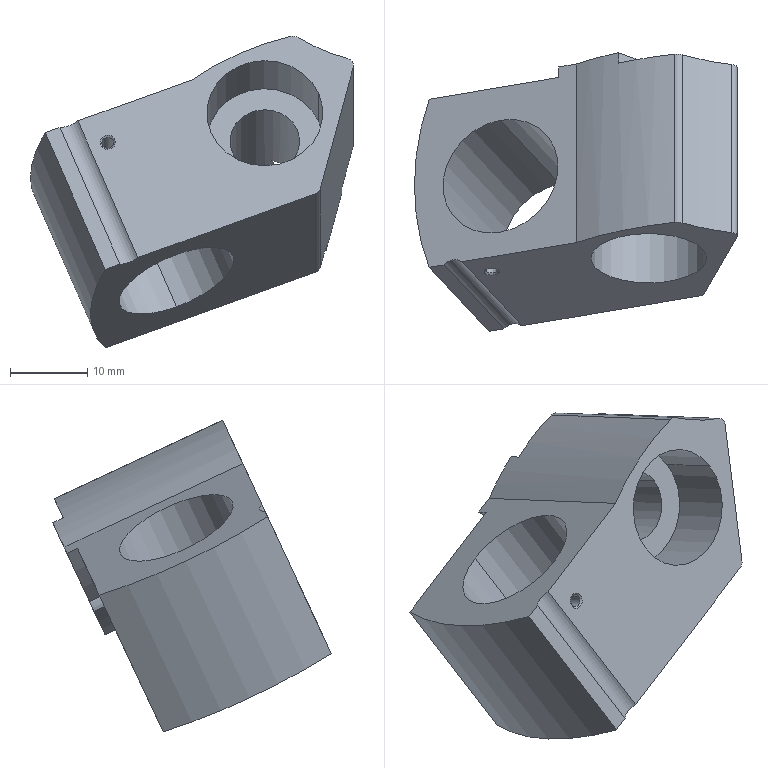Component | SolidWorks | 1369126_DSM_40_270_CC_HD_A_B_0-1_704066_DSM_40_BL_HZ-1 | 1 solid | 31 faces | box 41.79 x 36.01 x 40.31 mm | volume 12657 mm3 | cylinder 19 | plane 10 | cone 2 | commonest cylinder face diameters 16 x2 15 x2 9 x2 1.567 x2 61.3 x2 78.5 x2 2 x2 70 x1
STEP:
#1=COLOUR_RGB('',0.7922,0.8196,0.9333);
#2=FILL_AREA_STYLE_COLOUR('',#1);
#3=FILL_AREA_STYLE('',(#2));
#4=SURFACE_STYLE_FILL_AREA(#3);
#5=SURFACE_SIDE_STYLE('',(#4));
#6=SURFACE_STYLE_USAGE(.BOTH.,#5);
#7=PRESENTATION_STYLE_ASSIGNMENT((#6));
#8=CARTESIAN_POINT('',(-10.55,80.841,10.338));
#9=VERTEX_POINT('',#8);
#10=CARTESIAN_POINT('',(-10.55,81.412,10.072));
#11=VERTEX_POINT('',#10);
#12=CARTESIAN_POINT('',(-10.55,81.126,10.205));
#13=DIRECTION('',(-0.3689,0.3928,0.8424));
#14=DIRECTION('',(0.,0.9063,-0.4226));
#15=AXIS2_PLACEMENT_3D('',#12,#13,#14);
#16=CIRCLE('',#15,0.315);
#17=EDGE_CURVE('',#9,#11,#16,.T.);
#18=ORIENTED_EDGE('',*,*,#17,.T.);
#19=CARTESIAN_POINT('',(-10.245,81.087,9.375));
#20=VERTEX_POINT('',#19);
#21=CARTESIAN_POINT('',(-10.57,81.433,10.116));
#22=DIRECTION('',(0.3689,-0.3928,-0.8424));
#23=VECTOR('',#22,39.37);
#24=LINE('',#21,#23);
#25=EDGE_CURVE('',#11,#20,#24,.T.);
#26=ORIENTED_EDGE('',*,*,#25,.T.);
#27=CARTESIAN_POINT('',(-10.245,80.516,9.641));
#28=VERTEX_POINT('',#27);
#29=CARTESIAN_POINT('',(-10.245,80.802,9.508));
#30=DIRECTION('',(0.3689,-0.3928,-0.8424));
#31=DIRECTION('',(0.,-0.9063,0.4226));
#32=AXIS2_PLACEMENT_3D('',#29,#30,#31);
#33=CIRCLE('',#32,0.315);
#34=EDGE_CURVE('',#20,#28,#33,.T.);
#35=ORIENTED_EDGE('',*,*,#34,.T.);
#36=CARTESIAN_POINT('',(-10.57,80.862,10.382));
#37=DIRECTION('',(0.3689,-0.3928,-0.8424));
#38=VECTOR('',#37,39.37);
#39=LINE('',#36,#38);
#40=EDGE_CURVE('',#9,#28,#39,.T.);
#41=ORIENTED_EDGE('',*,*,#40,.F.);
#42=EDGE_LOOP('',(#18,#26,#35,#41));
#43=FACE_OUTER_BOUND('',#42,.T.);
#44=CARTESIAN_POINT('',(-10.57,81.147,10.249));
#45=DIRECTION('',(0.3689,-0.3928,-0.8424));
#46=DIRECTION('',(0.,-0.9063,0.4226));
#47=AXIS2_PLACEMENT_3D('',#44,#45,#46);
#48=CYLINDRICAL_SURFACE('',#47,0.315);
#49=ADVANCED_FACE('',(#43),#48,.F.);
#50=CARTESIAN_POINT('',(-10.566,80.652,10.22));
#51=VERTEX_POINT('',#50);
#52=CARTESIAN_POINT('',(-10.624,80.642,10.2));
#53=VERTEX_POINT('',#52);
#54=CARTESIAN_POINT('',(-10.595,80.647,10.21));
#55=DIRECTION('',(0.,-0.9063,0.4226));
#56=DIRECTION('',(-0.9295,-0.1559,-0.3344));
#57=AXIS2_PLACEMENT_3D('',#54,#55,#56);
#58=CIRCLE('',#57,0.03085);
#59=EDGE_CURVE('',#51,#53,#58,.T.);
#60=ORIENTED_EDGE('',*,*,#59,.F.);
#61=CARTESIAN_POINT('',(-10.558,80.646,10.227));
#62=VERTEX_POINT('',#61);
#63=CARTESIAN_POINT('',(-10.558,80.646,10.227));
#64=DIRECTION('',(0.6572,-0.5306,0.5353));
#65=VECTOR('',#64,39.37);
#66=LINE('',#63,#65);
#67=EDGE_CURVE('',#51,#62,#66,.T.);
#68=ORIENTED_EDGE('',*,*,#67,.T.);
#69=CARTESIAN_POINT('',(-10.631,80.633,10.2));
#70=VERTEX_POINT('',#69);
#71=CARTESIAN_POINT('',(-10.595,80.64,10.213));
#72=DIRECTION('',(0.,-0.9063,0.4226));
#73=DIRECTION('',(-0.9295,-0.1559,-0.3344));
#74=AXIS2_PLACEMENT_3D('',#71,#72,#73);
#75=CIRCLE('',#74,0.03937);
#76=EDGE_CURVE('',#62,#70,#75,.T.);
#77=ORIENTED_EDGE('',*,*,#76,.T.);
#78=CARTESIAN_POINT('',(-10.631,80.633,10.2));
#79=DIRECTION('',(-0.6572,-0.7511,0.0624));
#80=VECTOR('',#79,39.37);
#81=LINE('',#78,#80);
#82=EDGE_CURVE('',#53,#70,#81,.T.);
#83=ORIENTED_EDGE('',*,*,#82,.F.);
#84=EDGE_LOOP('',(#60,#68,#77,#83));
#85=FACE_OUTER_BOUND('',#84,.T.);
#86=CARTESIAN_POINT('',(-10.595,80.64,10.213));
#87=DIRECTION('',(0.,-0.9063,0.4226));
#88=DIRECTION('',(-0.9295,-0.1559,-0.3344));
#89=AXIS2_PLACEMENT_3D('',#86,#87,#88);
#90=CONICAL_SURFACE('',#89,0.03937,0.7854);
#91=ADVANCED_FACE('',(#85),#90,.F.);
#92=CARTESIAN_POINT('',(-9.521,81.061,10.317));
#93=VERTEX_POINT('',#92);
#94=CARTESIAN_POINT('',(-10.069,80.969,10.119));
#95=VERTEX_POINT('',#94);
#96=CARTESIAN_POINT('',(-9.795,81.015,10.218));
#97=DIRECTION('',(0.,-0.9063,0.4226));
#98=DIRECTION('',(-0.9295,-0.1559,-0.3344));
#99=AXIS2_PLACEMENT_3D('',#96,#97,#98);
#100=CIRCLE('',#99,0.2953);
#101=EDGE_CURVE('',#93,#95,#100,.T.);
#102=ORIENTED_EDGE('',*,*,#101,.F.);
#103=CARTESIAN_POINT('',(-9.521,80.755,10.46));
#104=VERTEX_POINT('',#103);
#105=CARTESIAN_POINT('',(-9.521,80.755,10.46));
#106=DIRECTION('',(0.,-0.9063,0.4226));
#107=VECTOR('',#106,39.37);
#108=LINE('',#105,#107);
#109=EDGE_CURVE('',#93,#104,#108,.T.);
#110=ORIENTED_EDGE('',*,*,#109,.T.);
#111=CARTESIAN_POINT('',(-10.069,80.662,10.263));
#112=VERTEX_POINT('',#111);
#113=CARTESIAN_POINT('',(-9.795,80.708,10.361));
#114=DIRECTION('',(0.,-0.9063,0.4226));
#115=DIRECTION('',(-0.9295,-0.1559,-0.3344));
#116=AXIS2_PLACEMENT_3D('',#113,#114,#115);
#117=CIRCLE('',#116,0.2953);
#118=EDGE_CURVE('',#104,#112,#117,.T.);
#119=ORIENTED_EDGE('',*,*,#118,.T.);
#120=CARTESIAN_POINT('',(-10.069,80.662,10.263));
#121=DIRECTION('',(0.,-0.9063,0.4226));
#122=VECTOR('',#121,39.37);
#123=LINE('',#120,#122);
#124=EDGE_CURVE('',#95,#112,#123,.T.);
#125=ORIENTED_EDGE('',*,*,#124,.F.);
#126=EDGE_LOOP('',(#102,#110,#119,#125));
#127=FACE_OUTER_BOUND('',#126,.T.);
#128=CARTESIAN_POINT('',(-9.795,80.708,10.361));
#129=DIRECTION('',(0.,-0.9063,0.4226));
#130=DIRECTION('',(-0.9295,-0.1559,-0.3344));
#131=AXIS2_PLACEMENT_3D('',#128,#129,#130);
#132=CYLINDRICAL_SURFACE('',#131,0.2953);
#133=ADVANCED_FACE('',(#127),#132,.F.);
#134=CARTESIAN_POINT('',(-9.63,81.646,9.996));
#135=VERTEX_POINT('',#134);
#136=CARTESIAN_POINT('',(-9.668,81.671,10.049));
#137=VERTEX_POINT('',#136);
#138=CARTESIAN_POINT('',(-9.795,81.618,9.937));
#139=DIRECTION('',(0.,-0.9063,0.4226));
#140=DIRECTION('',(-0.9295,-0.1559,-0.3344));
#141=AXIS2_PLACEMENT_3D('',#138,#139,#140);
#142=CIRCLE('',#141,0.1772);
#143=EDGE_CURVE('',#135,#137,#142,.T.);
#144=ORIENTED_EDGE('',*,*,#143,.F.);
#145=CARTESIAN_POINT('',(-9.63,81.043,10.277));
#146=VERTEX_POINT('',#145);
#147=CARTESIAN_POINT('',(-9.63,80.736,10.421));
#148=DIRECTION('',(0.,-0.9063,0.4226));
#149=VECTOR('',#148,39.37);
#150=LINE('',#147,#149);
#151=EDGE_CURVE('',#135,#146,#150,.T.);
#152=ORIENTED_EDGE('',*,*,#151,.T.);
#153=CARTESIAN_POINT('',(-9.96,80.988,10.159));
#154=VERTEX_POINT('',#153);
#155=CARTESIAN_POINT('',(-9.795,81.015,10.218));
#156=DIRECTION('',(0.,-0.9063,0.4226));
#157=DIRECTION('',(-0.9295,-0.1559,-0.3344));
#158=AXIS2_PLACEMENT_3D('',#155,#156,#157);
#159=CIRCLE('',#158,0.1772);
#160=EDGE_CURVE('',#146,#154,#159,.T.);
#161=ORIENTED_EDGE('',*,*,#160,.T.);
#162=CARTESIAN_POINT('',(-9.96,81.591,9.878));
#163=VERTEX_POINT('',#162);
#164=CARTESIAN_POINT('',(-9.96,80.681,10.302));
#165=DIRECTION('',(0.,-0.9063,0.4226));
#166=VECTOR('',#165,39.37);
#167=LINE('',#164,#166);
#168=EDGE_CURVE('',#163,#154,#167,.T.);
#169=ORIENTED_EDGE('',*,*,#168,.F.);
#170=CARTESIAN_POINT('',(-9.753,81.691,10.093));
#171=VERTEX_POINT('',#170);
#172=CARTESIAN_POINT('',(-9.795,81.618,9.937));
#173=DIRECTION('',(0.,-0.9063,0.4226));
#174=DIRECTION('',(-0.9295,-0.1559,-0.3344));
#175=AXIS2_PLACEMENT_3D('',#172,#173,#174);
#176=CIRCLE('',#175,0.1772);
#177=EDGE_CURVE('',#171,#163,#176,.T.);
#178=ORIENTED_EDGE('',*,*,#177,.F.);
#179=CARTESIAN_POINT('',(-9.753,81.638,10.118));
#180=VERTEX_POINT('',#179);
#181=CARTESIAN_POINT('',(-9.753,81.39,10.234));
#182=DIRECTION('',(0.,-0.9063,0.4226));
#183=VECTOR('',#182,39.37);
#184=LINE('',#181,#183);
#185=EDGE_CURVE('',#171,#180,#184,.T.);
#186=ORIENTED_EDGE('',*,*,#185,.T.);
#187=CARTESIAN_POINT('',(-9.668,81.617,10.074));
#188=VERTEX_POINT('',#187);
#189=CARTESIAN_POINT('',(-9.795,81.565,9.962));
#190=DIRECTION('',(0.,-0.9063,0.4226));
#191=DIRECTION('',(-0.9295,-0.1559,-0.3344));
#192=AXIS2_PLACEMENT_3D('',#189,#190,#191);
#193=CIRCLE('',#192,0.1772);
#194=EDGE_CURVE('',#188,#180,#193,.T.);
#195=ORIENTED_EDGE('',*,*,#194,.F.);
#196=CARTESIAN_POINT('',(-9.668,81.369,10.19));
#197=DIRECTION('',(-0.,0.9063,-0.4226));
#198=VECTOR('',#197,39.37);
#199=LINE('',#196,#198);
#200=EDGE_CURVE('',#188,#137,#199,.T.);
#201=ORIENTED_EDGE('',*,*,#200,.T.);
#202=EDGE_LOOP('',(#144,#152,#161,#169,#178,#186,#195,#201));
#203=FACE_OUTER_BOUND('',#202,.T.);
#204=CARTESIAN_POINT('',(-9.795,80.708,10.361));
#205=DIRECTION('',(0.,-0.9063,0.4226));
#206=DIRECTION('',(-0.9295,-0.1559,-0.3344));
#207=AXIS2_PLACEMENT_3D('',#204,#205,#206);
#208=CYLINDRICAL_SURFACE('',#207,0.1772);
#209=ADVANCED_FACE('',(#203),#208,.F.);
#210=CARTESIAN_POINT('',(-10.624,80.785,10.133));
#211=VERTEX_POINT('',#210);
#212=CARTESIAN_POINT('',(-10.566,80.772,10.164));
#213=VERTEX_POINT('',#212);
#214=CARTESIAN_POINT('',(-10.624,80.785,10.133));
#215=CARTESIAN_POINT('',(-10.625,80.786,10.137));
#216=CARTESIAN_POINT('',(-10.626,80.788,10.141));
#217=CARTESIAN_POINT('',(-10.626,80.79,10.149));
#218=CARTESIAN_POINT('',(-10.625,80.79,10.153));
#219=CARTESIAN_POINT('',(-10.62,80.791,10.165));
#220=CARTESIAN_POINT('',(-10.614,80.791,10.171));
#221=CARTESIAN_POINT('',(-10.599,80.788,10.179));
#222=CARTESIAN_POINT('',(-10.591,80.785,10.181));
#223=CARTESIAN_POINT('',(-10.58,80.781,10.178));
#224=CARTESIAN_POINT('',(-10.576,80.779,10.176));
#225=CARTESIAN_POINT('',(-10.57,80.776,10.171));
#226=CARTESIAN_POINT('',(-10.568,80.774,10.168));
#227=CARTESIAN_POINT('',(-10.566,80.772,10.164));
#228=B_SPLINE_CURVE_WITH_KNOTS('',3,(#214,#215,#216,#217,#218,#219,#220,#221,#222,#223,#224,#225,#226,#227),.UNSPECIFIED.,.F.,.F.,(4,2,2,2,2,2,4),(0.,0.0003181,0.0006361,0.001272,0.001908,0.002226,0.002544),.UNSPECIFIED.);
#229=EDGE_CURVE('',#211,#213,#228,.T.);
#230=ORIENTED_EDGE('',*,*,#229,.T.);
#231=CARTESIAN_POINT('',(-10.566,80.644,10.224));
#232=DIRECTION('',(0.,-0.9063,0.4226));
#233=VECTOR('',#232,39.37);
#234=LINE('',#231,#233);
#235=EDGE_CURVE('',#213,#51,#234,.T.);
#236=ORIENTED_EDGE('',*,*,#235,.T.);
#237=ORIENTED_EDGE('',*,*,#59,.T.);
#238=CARTESIAN_POINT('',(-10.624,80.635,10.203));
#239=DIRECTION('',(0.,-0.9063,0.4226));
#240=VECTOR('',#239,39.37);
#241=LINE('',#238,#240);
#242=EDGE_CURVE('',#211,#53,#241,.T.);
#243=ORIENTED_EDGE('',*,*,#242,.F.);
#244=EDGE_LOOP('',(#230,#236,#237,#243));
#245=FACE_OUTER_BOUND('',#244,.T.);
#246=CARTESIAN_POINT('',(-10.595,80.64,10.213));
#247=DIRECTION('',(0.,-0.9063,0.4226));
#248=DIRECTION('',(-0.9295,-0.1559,-0.3344));
#249=AXIS2_PLACEMENT_3D('',#246,#247,#248);
#250=CYLINDRICAL_SURFACE('',#249,0.03085);
#251=ADVANCED_FACE('',(#245),#250,.F.);
#252=ORIENTED_EDGE('',*,*,#235,.F.);
#253=CARTESIAN_POINT('',(-10.566,80.772,10.164));
#254=CARTESIAN_POINT('',(-10.565,80.771,10.161));
#255=CARTESIAN_POINT('',(-10.564,80.769,10.157));
#256=CARTESIAN_POINT('',(-10.564,80.767,10.149));
#257=CARTESIAN_POINT('',(-10.565,80.765,10.145));
#258=CARTESIAN_POINT('',(-10.57,80.763,10.133));
#259=CARTESIAN_POINT('',(-10.577,80.763,10.127));
#260=CARTESIAN_POINT('',(-10.591,80.766,10.119));
#261=CARTESIAN_POINT('',(-10.599,80.77,10.118));
#262=CARTESIAN_POINT('',(-10.61,80.775,10.121));
#263=CARTESIAN_POINT('',(-10.614,80.777,10.122));
#264=CARTESIAN_POINT('',(-10.62,80.781,10.127));
#265=CARTESIAN_POINT('',(-10.622,80.783,10.13));
#266=CARTESIAN_POINT('',(-10.624,80.785,10.133));
#267=B_SPLINE_CURVE_WITH_KNOTS('',3,(#253,#254,#255,#256,#257,#258,#259,#260,#261,#262,#263,#264,#265,#266),.UNSPECIFIED.,.F.,.F.,(4,2,2,2,2,2,4),(0.002544,0.002862,0.00318,0.003816,0.004452,0.00477,0.005088),.UNSPECIFIED.);
#268=EDGE_CURVE('',#213,#211,#267,.T.);
#269=ORIENTED_EDGE('',*,*,#268,.T.);
#270=ORIENTED_EDGE('',*,*,#242,.T.);
#271=CARTESIAN_POINT('',(-10.595,80.647,10.21));
#272=DIRECTION('',(0.,-0.9063,0.4226));
#273=DIRECTION('',(-0.9295,-0.1559,-0.3344));
#274=AXIS2_PLACEMENT_3D('',#271,#272,#273);
#275=CIRCLE('',#274,0.03085);
#276=EDGE_CURVE('',#53,#51,#275,.T.);
#277=ORIENTED_EDGE('',*,*,#276,.T.);
#278=EDGE_LOOP('',(#252,#269,#270,#277));
#279=FACE_OUTER_BOUND('',#278,.T.);
#280=CARTESIAN_POINT('',(-10.595,80.64,10.213));
#281=DIRECTION('',(0.,-0.9063,0.4226));
#282=DIRECTION('',(-0.9295,-0.1559,-0.3344));
#283=AXIS2_PLACEMENT_3D('',#280,#281,#282);
#284=CYLINDRICAL_SURFACE('',#283,0.03085);
#285=ADVANCED_FACE('',(#279),#284,.F.);
#286=CARTESIAN_POINT('',(-9.83,81.545,9.78));
#287=VERTEX_POINT('',#286);
#288=CARTESIAN_POINT('',(-9.483,81.489,9.661));
#289=VERTEX_POINT('',#288);
#290=CARTESIAN_POINT('',(-9.114,82.124,11.021));
#291=DIRECTION('',(0.,-0.9063,0.4226));
#292=DIRECTION('',(-0.9295,-0.1559,-0.3344));
#293=AXIS2_PLACEMENT_3D('',#290,#291,#292);
#294=CIRCLE('',#293,1.545);
#295=EDGE_CURVE('',#287,#289,#294,.T.);
#296=ORIENTED_EDGE('',*,*,#295,.F.);
#297=CARTESIAN_POINT('',(-9.795,81.618,9.937));
#298=DIRECTION('',(0.,-0.9063,0.4226));
#299=DIRECTION('',(-0.9295,-0.1559,-0.3344));
#300=AXIS2_PLACEMENT_3D('',#297,#298,#299);
#301=CIRCLE('',#300,0.1772);
#302=EDGE_CURVE('',#287,#135,#301,.T.);
#303=ORIENTED_EDGE('',*,*,#302,.T.);
#304=ORIENTED_EDGE('',*,*,#143,.T.);
#305=CARTESIAN_POINT('',(-9.402,81.628,9.959));
#306=VERTEX_POINT('',#305);
#307=CARTESIAN_POINT('',(-9.114,82.124,11.021));
#308=DIRECTION('',(-0.,0.9063,-0.4226));
#309=DIRECTION('',(-0.9295,-0.1559,-0.3344));
#310=AXIS2_PLACEMENT_3D('',#307,#308,#309);
#311=CIRCLE('',#310,1.207);
#312=EDGE_CURVE('',#306,#137,#311,.T.);
#313=ORIENTED_EDGE('',*,*,#312,.F.);
#314=CARTESIAN_POINT('',(-9.513,81.439,9.552));
#315=DIRECTION('',(0.2387,0.4104,0.8801));
#316=VECTOR('',#315,39.37);
#317=LINE('',#314,#316);
#318=EDGE_CURVE('',#289,#306,#317,.T.);
#319=ORIENTED_EDGE('',*,*,#318,.F.);
#320=EDGE_LOOP('',(#296,#303,#304,#313,#319));
#321=FACE_OUTER_BOUND('',#320,.T.);
#322=CARTESIAN_POINT('',(-9.382,81.732,10.181));
#323=DIRECTION('',(0.,-0.9063,0.4226));
#324=DIRECTION('',(-0.9295,-0.1559,-0.3344));
#325=AXIS2_PLACEMENT_3D('',#322,#323,#324);
#326=PLANE('',#325);
#327=ADVANCED_FACE('',(#321),#326,.F.);
#328=ORIENTED_EDGE('',*,*,#200,.F.);
#329=CARTESIAN_POINT('',(-9.402,81.575,9.984));
#330=VERTEX_POINT('',#329);
#331=CARTESIAN_POINT('',(-9.114,82.07,11.046));
#332=DIRECTION('',(-0.,0.9063,-0.4226));
#333=DIRECTION('',(0.9295,0.1559,0.3344));
#334=AXIS2_PLACEMENT_3D('',#331,#332,#333);
#335=CIRCLE('',#334,1.207);
#336=EDGE_CURVE('',#330,#188,#335,.T.);
#337=ORIENTED_EDGE('',*,*,#336,.F.);
#338=CARTESIAN_POINT('',(-9.402,81.628,9.959));
#339=DIRECTION('',(0.,-0.9063,0.4226));
#340=VECTOR('',#339,39.37);
#341=LINE('',#338,#340);
#342=EDGE_CURVE('',#306,#330,#341,.T.);
#343=ORIENTED_EDGE('',*,*,#342,.F.);
#344=ORIENTED_EDGE('',*,*,#312,.T.);
#345=EDGE_LOOP('',(#328,#337,#343,#344));
#346=FACE_OUTER_BOUND('',#345,.T.);
#347=CARTESIAN_POINT('',(-9.114,82.124,11.021));
#348=DIRECTION('',(0.,-0.9063,0.4226));
#349=DIRECTION('',(-0.9295,-0.1559,-0.3344));
#350=AXIS2_PLACEMENT_3D('',#347,#348,#349);
#351=CYLINDRICAL_SURFACE('',#350,1.207);
#352=ADVANCED_FACE('',(#346),#351,.F.);
#353=CARTESIAN_POINT('',(-9.83,81.491,9.805));
#354=VERTEX_POINT('',#353);
#355=CARTESIAN_POINT('',(-9.83,81.243,9.92));
#356=DIRECTION('',(0.,-0.9063,0.4226));
#357=VECTOR('',#356,39.37);
#358=LINE('',#355,#357);
#359=EDGE_CURVE('',#287,#354,#358,.T.);
#360=ORIENTED_EDGE('',*,*,#359,.F.);
#361=ORIENTED_EDGE('',*,*,#295,.T.);
#362=CARTESIAN_POINT('',(-9.483,81.436,9.686));
#363=VERTEX_POINT('',#362);
#364=CARTESIAN_POINT('',(-9.483,81.489,9.661));
#365=DIRECTION('',(-0.,0.9063,-0.4226));
#366=VECTOR('',#365,39.37);
#367=LINE('',#364,#366);
#368=EDGE_CURVE('',#363,#289,#367,.T.);
#369=ORIENTED_EDGE('',*,*,#368,.F.);
#370=CARTESIAN_POINT('',(-9.114,82.07,11.046));
#371=DIRECTION('',(0.,-0.9063,0.4226));
#372=DIRECTION('',(-0.9295,-0.1559,-0.3344));
#373=AXIS2_PLACEMENT_3D('',#370,#371,#372);
#374=CIRCLE('',#373,1.545);
#375=EDGE_CURVE('',#354,#363,#374,.T.);
#376=ORIENTED_EDGE('',*,*,#375,.F.);
#377=EDGE_LOOP('',(#360,#361,#369,#376));
#378=FACE_OUTER_BOUND('',#377,.T.);
#379=CARTESIAN_POINT('',(-9.114,82.124,11.021));
#380=DIRECTION('',(0.,-0.9063,0.4226));
#381=DIRECTION('',(-0.9295,-0.1559,-0.3344));
#382=AXIS2_PLACEMENT_3D('',#379,#380,#381);
#383=CYLINDRICAL_SURFACE('',#382,1.545);
#384=ADVANCED_FACE('',(#378),#383,.T.);
#385=CARTESIAN_POINT('',(-9.949,81.755,10.231));
#386=VERTEX_POINT('',#385);
#387=CARTESIAN_POINT('',(-9.114,82.124,11.021));
#388=DIRECTION('',(-0.,0.9063,-0.4226));
#389=DIRECTION('',(-0.9295,-0.1559,-0.3344));
#390=AXIS2_PLACEMENT_3D('',#387,#388,#389);
#391=CIRCLE('',#390,1.207);
#392=EDGE_CURVE('',#171,#386,#391,.T.);
#393=ORIENTED_EDGE('',*,*,#392,.F.);
#394=ORIENTED_EDGE('',*,*,#177,.T.);
#395=CARTESIAN_POINT('',(-9.926,81.568,9.829));
#396=VERTEX_POINT('',#395);
#397=CARTESIAN_POINT('',(-9.795,81.618,9.937));
#398=DIRECTION('',(0.,-0.9063,0.4226));
#399=DIRECTION('',(-0.9295,-0.1559,-0.3344));
#400=AXIS2_PLACEMENT_3D('',#397,#398,#399);
#401=CIRCLE('',#400,0.1772);
#402=EDGE_CURVE('',#163,#396,#401,.T.);
#403=ORIENTED_EDGE('',*,*,#402,.T.);
#404=CARTESIAN_POINT('',(-10.254,81.683,10.075));
#405=VERTEX_POINT('',#404);
#406=CARTESIAN_POINT('',(-9.114,82.124,11.021));
#407=DIRECTION('',(0.,-0.9063,0.4226));
#408=DIRECTION('',(-0.9295,-0.1559,-0.3344));
#409=AXIS2_PLACEMENT_3D('',#406,#407,#408);
#410=CIRCLE('',#409,1.545);
#411=EDGE_CURVE('',#405,#396,#410,.T.);
#412=ORIENTED_EDGE('',*,*,#411,.F.);
#413=CARTESIAN_POINT('',(-10.164,81.698,10.107));
#414=VERTEX_POINT('',#413);
#415=CARTESIAN_POINT('',(-10.164,81.698,10.107));
#416=DIRECTION('',(-0.9295,-0.1559,-0.3344));
#417=VECTOR('',#416,39.37);
#418=LINE('',#415,#417);
#419=EDGE_CURVE('',#414,#405,#418,.T.);
#420=ORIENTED_EDGE('',*,*,#419,.F.);
#421=CARTESIAN_POINT('',(-9.324,81.236,9.118));
#422=DIRECTION('',(0.,-0.9063,0.4226));
#423=DIRECTION('',(-0.9295,-0.1559,-0.3344));
#424=AXIS2_PLACEMENT_3D('',#421,#422,#423);
#425=CIRCLE('',#424,1.378);
#426=EDGE_CURVE('',#386,#414,#425,.T.);
#427=ORIENTED_EDGE('',*,*,#426,.F.);
#428=EDGE_LOOP('',(#393,#394,#403,#412,#420,#427));
#429=FACE_OUTER_BOUND('',#428,.T.);
#430=CARTESIAN_POINT('',(-9.382,81.732,10.181));
#431=DIRECTION('',(0.,-0.9063,0.4226));
#432=DIRECTION('',(-0.9295,-0.1559,-0.3344));
#433=AXIS2_PLACEMENT_3D('',#430,#431,#432);
#434=PLANE('',#433);
#435=ADVANCED_FACE('',(#429),#434,.F.);
#436=CARTESIAN_POINT('',(-10.913,80.662,10.262));
#437=VERTEX_POINT('',#436);
#438=CARTESIAN_POINT('',(-10.608,80.338,9.566));
#439=VERTEX_POINT('',#438);
#440=CARTESIAN_POINT('',(-11.016,80.772,10.498));
#441=DIRECTION('',(0.3689,-0.3928,-0.8424));
#442=VECTOR('',#441,39.37);
#443=LINE('',#440,#442);
#444=EDGE_CURVE('',#437,#439,#443,.T.);
#445=ORIENTED_EDGE('',*,*,#444,.T.);
#446=CARTESIAN_POINT('',(-10.533,80.35,9.593));
#447=VERTEX_POINT('',#446);
#448=CARTESIAN_POINT('',(-10.725,80.318,9.524));
#449=DIRECTION('',(0.9295,0.1559,0.3344));
#450=VECTOR('',#449,39.37);
#451=LINE('',#448,#450);
#452=EDGE_CURVE('',#439,#447,#451,.T.);
#453=ORIENTED_EDGE('',*,*,#452,.T.);
#454=CARTESIAN_POINT('',(-10.838,80.675,10.289));
#455=VERTEX_POINT('',#454);
#456=CARTESIAN_POINT('',(-10.941,80.785,10.525));
#457=DIRECTION('',(0.3689,-0.3928,-0.8424));
#458=VECTOR('',#457,39.37);
#459=LINE('',#456,#458);
#460=EDGE_CURVE('',#455,#447,#459,.T.);
#461=ORIENTED_EDGE('',*,*,#460,.F.);
#462=CARTESIAN_POINT('',(-10.164,80.788,10.532));
#463=DIRECTION('',(-0.9295,-0.1559,-0.3344));
#464=VECTOR('',#463,39.37);
#465=LINE('',#462,#464);
#466=EDGE_CURVE('',#455,#437,#465,.T.);
#467=ORIENTED_EDGE('',*,*,#466,.T.);
#468=EDGE_LOOP('',(#445,#453,#461,#467));
#469=FACE_OUTER_BOUND('',#468,.T.);
#470=CARTESIAN_POINT('',(-9.382,80.822,10.605));
#471=DIRECTION('',(0.,-0.9063,0.4226));
#472=DIRECTION('',(-0.9295,-0.1559,-0.3344));
#473=AXIS2_PLACEMENT_3D('',#470,#471,#472);
#474=PLANE('',#473);
#475=ADVANCED_FACE('',(#469),#474,.T.);
#476=CARTESIAN_POINT('',(-9.372,81.695,10.24));
#477=VERTEX_POINT('',#476);
#478=CARTESIAN_POINT('',(-9.344,81.675,10.197));
#479=VERTEX_POINT('',#478);
#480=CARTESIAN_POINT('',(-9.382,81.679,10.206));
#481=DIRECTION('',(-0.,0.9063,-0.4226));
#482=DIRECTION('',(-0.9295,-0.1559,-0.3344));
#483=AXIS2_PLACEMENT_3D('',#480,#481,#482);
#484=CIRCLE('',#483,0.03937);
#485=EDGE_CURVE('',#477,#479,#484,.T.);
#486=ORIENTED_EDGE('',*,*,#485,.F.);
#487=CARTESIAN_POINT('',(-9.372,80.838,10.64));
#488=VERTEX_POINT('',#487);
#489=CARTESIAN_POINT('',(-9.372,81.748,10.215));
#490=DIRECTION('',(0.,-0.9063,0.4226));
#491=VECTOR('',#490,39.37);
#492=LINE('',#489,#491);
#493=EDGE_CURVE('',#477,#488,#492,.T.);
#494=ORIENTED_EDGE('',*,*,#493,.T.);
#495=CARTESIAN_POINT('',(-9.344,80.818,10.597));
#496=VERTEX_POINT('',#495);
#497=CARTESIAN_POINT('',(-9.382,80.822,10.605));
#498=DIRECTION('',(0.,-0.9063,0.4226));
#499=DIRECTION('',(-0.9295,-0.1559,-0.3344));
#500=AXIS2_PLACEMENT_3D('',#497,#498,#499);
#501=CIRCLE('',#500,0.03937);
#502=EDGE_CURVE('',#496,#488,#501,.T.);
#503=ORIENTED_EDGE('',*,*,#502,.F.);
#504=CARTESIAN_POINT('',(-9.344,81.728,10.172));
#505=DIRECTION('',(0.,-0.9063,0.4226));
#506=VECTOR('',#505,39.37);
#507=LINE('',#504,#506);
#508=EDGE_CURVE('',#479,#496,#507,.T.);
#509=ORIENTED_EDGE('',*,*,#508,.F.);
#510=EDGE_LOOP('',(#486,#494,#503,#509));
#511=FACE_OUTER_BOUND('',#510,.T.);
#512=CARTESIAN_POINT('',(-9.382,81.732,10.181));
#513=DIRECTION('',(0.,-0.9063,0.4226));
#514=DIRECTION('',(-0.9295,-0.1559,-0.3344));
#515=AXIS2_PLACEMENT_3D('',#512,#513,#514);
#516=CYLINDRICAL_SURFACE('',#515,0.03937);
#517=ADVANCED_FACE('',(#511),#516,.T.);
#518=CARTESIAN_POINT('',(-9.513,81.385,9.577));
#519=DIRECTION('',(-0.2387,-0.4104,-0.8801));
#520=VECTOR('',#519,39.37);
#521=LINE('',#518,#520);
#522=EDGE_CURVE('',#479,#330,#521,.T.);
#523=ORIENTED_EDGE('',*,*,#522,.F.);
#524=ORIENTED_EDGE('',*,*,#508,.T.);
#525=CARTESIAN_POINT('',(-9.513,80.529,9.976));
#526=VERTEX_POINT('',#525);
#527=CARTESIAN_POINT('',(-9.513,80.529,9.976));
#528=DIRECTION('',(0.2387,0.4104,0.8801));
#529=VECTOR('',#528,39.37);
#530=LINE('',#527,#529);
#531=EDGE_CURVE('',#526,#496,#530,.T.);
#532=ORIENTED_EDGE('',*,*,#531,.F.);
#533=CARTESIAN_POINT('',(-9.513,81.385,9.577));
#534=VERTEX_POINT('',#533);
#535=CARTESIAN_POINT('',(-9.513,81.439,9.552));
#536=DIRECTION('',(0.,-0.9063,0.4226));
#537=VECTOR('',#536,39.37);
#538=LINE('',#535,#537);
#539=EDGE_CURVE('',#534,#526,#538,.T.);
#540=ORIENTED_EDGE('',*,*,#539,.F.);
#541=CARTESIAN_POINT('',(-9.513,81.385,9.577));
#542=DIRECTION('',(-0.2387,-0.4104,-0.8801));
#543=VECTOR('',#542,39.37);
#544=LINE('',#541,#543);
#545=EDGE_CURVE('',#363,#534,#544,.T.);
#546=ORIENTED_EDGE('',*,*,#545,.F.);
#547=ORIENTED_EDGE('',*,*,#368,.T.);
#548=ORIENTED_EDGE('',*,*,#318,.T.);
#549=ORIENTED_EDGE('',*,*,#342,.T.);
#550=EDGE_LOOP('',(#523,#524,#532,#540,#546,#547,#548,#549));
#551=FACE_OUTER_BOUND('',#550,.T.);
#552=CARTESIAN_POINT('',(-9.513,81.439,9.552));
#553=DIRECTION('',(0.9711,-0.1009,-0.2163));
#554=DIRECTION('',(0.2387,0.4104,0.8801));
#555=AXIS2_PLACEMENT_3D('',#552,#553,#554);
#556=PLANE('',#555);
#557=ADVANCED_FACE('',(#551),#556,.T.);
#558=CARTESIAN_POINT('',(-9.536,81.374,9.552));
#559=VERTEX_POINT('',#558);
#560=CARTESIAN_POINT('',(-9.551,81.389,9.585));
#561=DIRECTION('',(-0.,0.9063,-0.4226));
#562=DIRECTION('',(-0.9295,-0.1559,-0.3344));
#563=AXIS2_PLACEMENT_3D('',#560,#561,#562);
#564=CIRCLE('',#563,0.03937);
#565=EDGE_CURVE('',#534,#559,#564,.T.);
#566=ORIENTED_EDGE('',*,*,#565,.F.);
#567=ORIENTED_EDGE('',*,*,#539,.T.);
#568=CARTESIAN_POINT('',(-9.536,80.517,9.951));
#569=VERTEX_POINT('',#568);
#570=CARTESIAN_POINT('',(-9.551,80.533,9.984));
#571=DIRECTION('',(0.,-0.9063,0.4226));
#572=DIRECTION('',(-0.9295,-0.1559,-0.3344));
#573=AXIS2_PLACEMENT_3D('',#570,#571,#572);
#574=CIRCLE('',#573,0.03937);
#575=EDGE_CURVE('',#569,#526,#574,.T.);
#576=ORIENTED_EDGE('',*,*,#575,.F.);
#577=CARTESIAN_POINT('',(-9.536,81.427,9.527));
#578=DIRECTION('',(0.,-0.9063,0.4226));
#579=VECTOR('',#578,39.37);
#580=LINE('',#577,#579);
#581=EDGE_CURVE('',#559,#569,#580,.T.);
#582=ORIENTED_EDGE('',*,*,#581,.F.);
#583=EDGE_LOOP('',(#566,#567,#576,#582));
#584=FACE_OUTER_BOUND('',#583,.T.);
#585=CARTESIAN_POINT('',(-9.551,81.443,9.56));
#586=DIRECTION('',(0.,-0.9063,0.4226));
#587=DIRECTION('',(-0.9295,-0.1559,-0.3344));
#588=AXIS2_PLACEMENT_3D('',#585,#586,#587);
#589=CYLINDRICAL_SURFACE('',#588,0.03937);
#590=ADVANCED_FACE('',(#584),#589,.T.);
#591=CARTESIAN_POINT('',(-10.245,80.802,9.508));
#592=DIRECTION('',(0.3689,-0.3928,-0.8424));
#593=DIRECTION('',(0.,-0.9063,0.4226));
#594=AXIS2_PLACEMENT_3D('',#591,#592,#593);
#595=CIRCLE('',#594,0.315);
#596=EDGE_CURVE('',#28,#20,#595,.T.);
#597=ORIENTED_EDGE('',*,*,#596,.F.);
#598=ORIENTED_EDGE('',*,*,#34,.F.);
#599=EDGE_LOOP('',(#597,#598));
#600=FACE_BOUND('',#599,.T.);
#601=CARTESIAN_POINT('',(-10.608,81.194,9.166));
#602=VERTEX_POINT('',#601);
#603=CARTESIAN_POINT('',(-9.366,80.974,9.813));
#604=DIRECTION('',(-0.3689,0.3928,0.8424));
#605=DIRECTION('',(-0.,-0.9063,0.4226));
#606=AXIS2_PLACEMENT_3D('',#603,#604,#605);
#607=CIRCLE('',#606,1.417);
#608=EDGE_CURVE('',#602,#439,#607,.T.);
#609=ORIENTED_EDGE('',*,*,#608,.F.);
#610=CARTESIAN_POINT('',(-10.725,81.174,9.124));
#611=DIRECTION('',(-0.9295,-0.1559,-0.3344));
#612=VECTOR('',#611,39.37);
#613=LINE('',#610,#612);
#614=EDGE_CURVE('',#559,#602,#613,.T.);
#615=ORIENTED_EDGE('',*,*,#614,.F.);
#616=ORIENTED_EDGE('',*,*,#581,.T.);
#617=CARTESIAN_POINT('',(-10.442,80.365,9.626));
#618=VERTEX_POINT('',#617);
#619=CARTESIAN_POINT('',(-10.725,80.318,9.524));
#620=DIRECTION('',(0.9295,0.1559,0.3344));
#621=VECTOR('',#620,39.37);
#622=LINE('',#619,#621);
#623=EDGE_CURVE('',#618,#569,#622,.T.);
#624=ORIENTED_EDGE('',*,*,#623,.F.);
#625=CARTESIAN_POINT('',(-10.487,80.311,9.631));
#626=DIRECTION('',(0.3689,-0.3928,-0.8424));
#627=DIRECTION('',(0.,-0.9063,0.4226));
#628=AXIS2_PLACEMENT_3D('',#625,#626,#627);
#629=CIRCLE('',#628,0.07087);
#630=EDGE_CURVE('',#447,#618,#629,.T.);
#631=ORIENTED_EDGE('',*,*,#630,.F.);
#632=ORIENTED_EDGE('',*,*,#452,.F.);
#633=EDGE_LOOP('',(#609,#615,#616,#624,#631,#632));
#634=FACE_OUTER_BOUND('',#633,.T.);
#635=CARTESIAN_POINT('',(-10.725,81.228,9.099));
#636=DIRECTION('',(0.3689,-0.3928,-0.8424));
#637=DIRECTION('',(0.,-0.9063,0.4226));
#638=AXIS2_PLACEMENT_3D('',#635,#636,#637);
#639=PLANE('',#638);
#640=ADVANCED_FACE('',(#600,#634),#639,.T.);
#641=ORIENTED_EDGE('',*,*,#17,.F.);
#642=CARTESIAN_POINT('',(-10.55,81.126,10.205));
#643=DIRECTION('',(-0.3689,0.3928,0.8424));
#644=DIRECTION('',(0.,0.9063,-0.4226));
#645=AXIS2_PLACEMENT_3D('',#642,#643,#644);
#646=CIRCLE('',#645,0.315);
#647=EDGE_CURVE('',#11,#9,#646,.T.);
#648=ORIENTED_EDGE('',*,*,#647,.F.);
#649=EDGE_LOOP('',(#641,#648));
#650=FACE_BOUND('',#649,.T.);
#651=CARTESIAN_POINT('',(-10.913,81.519,9.863));
#652=VERTEX_POINT('',#651);
#653=CARTESIAN_POINT('',(-9.671,81.299,10.509));
#654=DIRECTION('',(0.3689,-0.3928,-0.8424));
#655=DIRECTION('',(0.,0.9063,-0.4226));
#656=AXIS2_PLACEMENT_3D('',#653,#654,#655);
#657=CIRCLE('',#656,1.417);
#658=EDGE_CURVE('',#437,#652,#657,.T.);
#659=ORIENTED_EDGE('',*,*,#658,.F.);
#660=ORIENTED_EDGE('',*,*,#466,.F.);
#661=CARTESIAN_POINT('',(-10.747,80.69,10.322));
#662=VERTEX_POINT('',#661);
#663=CARTESIAN_POINT('',(-10.792,80.636,10.327));
#664=DIRECTION('',(-0.3689,0.3928,0.8424));
#665=DIRECTION('',(0.,0.9063,-0.4226));
#666=AXIS2_PLACEMENT_3D('',#663,#664,#665);
#667=CIRCLE('',#666,0.07087);
#668=EDGE_CURVE('',#662,#455,#667,.T.);
#669=ORIENTED_EDGE('',*,*,#668,.F.);
#670=CARTESIAN_POINT('',(-10.164,80.788,10.532));
#671=VERTEX_POINT('',#670);
#672=CARTESIAN_POINT('',(-10.164,80.788,10.532));
#673=DIRECTION('',(-0.9295,-0.1559,-0.3344));
#674=VECTOR('',#673,39.37);
#675=LINE('',#672,#674);
#676=EDGE_CURVE('',#671,#662,#675,.T.);
#677=ORIENTED_EDGE('',*,*,#676,.F.);
#678=CARTESIAN_POINT('',(-10.164,81.698,10.107));
#679=DIRECTION('',(0.,-0.9063,0.4226));
#680=VECTOR('',#679,39.37);
#681=LINE('',#678,#680);
#682=EDGE_CURVE('',#414,#671,#681,.T.);
#683=ORIENTED_EDGE('',*,*,#682,.F.);
#684=ORIENTED_EDGE('',*,*,#419,.T.);
#685=CARTESIAN_POINT('',(-10.254,81.629,10.1));
#686=VERTEX_POINT('',#685);
#687=CARTESIAN_POINT('',(-10.254,81.683,10.075));
#688=DIRECTION('',(0.,-0.9063,0.4226));
#689=VECTOR('',#688,39.37);
#690=LINE('',#687,#689);
#691=EDGE_CURVE('',#405,#686,#690,.T.);
#692=ORIENTED_EDGE('',*,*,#691,.T.);
#693=CARTESIAN_POINT('',(-10.164,81.644,10.132));
#694=DIRECTION('',(0.9295,0.1559,0.3344));
#695=VECTOR('',#694,39.37);
#696=LINE('',#693,#695);
#697=EDGE_CURVE('',#652,#686,#696,.T.);
#698=ORIENTED_EDGE('',*,*,#697,.F.);
#699=EDGE_LOOP('',(#659,#660,#669,#677,#683,#684,#692,#698));
#700=FACE_OUTER_BOUND('',#699,.T.);
#701=CARTESIAN_POINT('',(-10.164,81.698,10.107));
#702=DIRECTION('',(-0.3689,0.3928,0.8424));
#703=DIRECTION('',(-0.,0.9063,-0.4226));
#704=AXIS2_PLACEMENT_3D('',#701,#702,#703);
#705=PLANE('',#704);
#706=ADVANCED_FACE('',(#650,#700),#705,.T.);
#707=CARTESIAN_POINT('',(-9.949,81.702,10.256));
#708=VERTEX_POINT('',#707);
#709=CARTESIAN_POINT('',(-9.664,81.747,10.353));
#710=VERTEX_POINT('',#709);
#711=CARTESIAN_POINT('',(-9.324,81.183,9.143));
#712=DIRECTION('',(-0.,0.9063,-0.4226));
#713=DIRECTION('',(-0.9295,-0.1559,-0.3344));
#714=AXIS2_PLACEMENT_3D('',#711,#712,#713);
#715=CIRCLE('',#714,1.378);
#716=EDGE_CURVE('',#708,#710,#715,.T.);
#717=ORIENTED_EDGE('',*,*,#716,.F.);
#718=CARTESIAN_POINT('',(-9.949,81.755,10.231));
#719=DIRECTION('',(0.,-0.9063,0.4226));
#720=VECTOR('',#719,39.37);
#721=LINE('',#718,#720);
#722=EDGE_CURVE('',#386,#708,#721,.T.);
#723=ORIENTED_EDGE('',*,*,#722,.F.);
#724=ORIENTED_EDGE('',*,*,#426,.T.);
#725=ORIENTED_EDGE('',*,*,#682,.T.);
#726=CARTESIAN_POINT('',(-9.664,80.891,10.752));
#727=VERTEX_POINT('',#726);
#728=CARTESIAN_POINT('',(-9.324,80.326,9.542));
#729=DIRECTION('',(0.,-0.9063,0.4226));
#730=DIRECTION('',(-0.9295,-0.1559,-0.3344));
#731=AXIS2_PLACEMENT_3D('',#728,#729,#730);
#732=CIRCLE('',#731,1.378);
#733=EDGE_CURVE('',#727,#671,#732,.T.);
#734=ORIENTED_EDGE('',*,*,#733,.F.);
#735=CARTESIAN_POINT('',(-9.664,81.801,10.328));
#736=DIRECTION('',(0.,-0.9063,0.4226));
#737=VECTOR('',#736,39.37);
#738=LINE('',#735,#737);
#739=EDGE_CURVE('',#710,#727,#738,.T.);
#740=ORIENTED_EDGE('',*,*,#739,.F.);
#741=EDGE_LOOP('',(#717,#723,#724,#725,#734,#740));
#742=FACE_OUTER_BOUND('',#741,.T.);
#743=CARTESIAN_POINT('',(-9.324,81.236,9.118));
#744=DIRECTION('',(0.,-0.9063,0.4226));
#745=DIRECTION('',(-0.9295,-0.1559,-0.3344));
#746=AXIS2_PLACEMENT_3D('',#743,#744,#745);
#747=CYLINDRICAL_SURFACE('',#746,1.378);
#748=ADVANCED_FACE('',(#742),#747,.T.);
#749=CARTESIAN_POINT('',(-9.626,81.744,10.347));
#750=VERTEX_POINT('',#749);
#751=CARTESIAN_POINT('',(-9.652,81.728,10.311));
#752=DIRECTION('',(-0.,0.9063,-0.4226));
#753=DIRECTION('',(-0.9295,-0.1559,-0.3344));
#754=AXIS2_PLACEMENT_3D('',#751,#752,#753);
#755=CIRCLE('',#754,0.04724);
#756=EDGE_CURVE('',#710,#750,#755,.T.);
#757=ORIENTED_EDGE('',*,*,#756,.F.);
#758=ORIENTED_EDGE('',*,*,#739,.T.);
#759=CARTESIAN_POINT('',(-9.626,80.888,10.746));
#760=VERTEX_POINT('',#759);
#761=CARTESIAN_POINT('',(-9.652,80.871,10.711));
#762=DIRECTION('',(0.,-0.9063,0.4226));
#763=DIRECTION('',(-0.9295,-0.1559,-0.3344));
#764=AXIS2_PLACEMENT_3D('',#761,#762,#763);
#765=CIRCLE('',#764,0.04724);
#766=EDGE_CURVE('',#760,#727,#765,.T.);
#767=ORIENTED_EDGE('',*,*,#766,.F.);
#768=CARTESIAN_POINT('',(-9.626,81.798,10.322));
#769=DIRECTION('',(0.,-0.9063,0.4226));
#770=VECTOR('',#769,39.37);
#771=LINE('',#768,#770);
#772=EDGE_CURVE('',#750,#760,#771,.T.);
#773=ORIENTED_EDGE('',*,*,#772,.F.);
#774=EDGE_LOOP('',(#757,#758,#767,#773));
#775=FACE_OUTER_BOUND('',#774,.T.);
#776=CARTESIAN_POINT('',(-9.652,81.781,10.286));
#777=DIRECTION('',(0.,-0.9063,0.4226));
#778=DIRECTION('',(-0.9295,-0.1559,-0.3344));
#779=AXIS2_PLACEMENT_3D('',#776,#777,#778);
#780=CYLINDRICAL_SURFACE('',#779,0.04724);
#781=ADVANCED_FACE('',(#775),#780,.T.);
#782=CARTESIAN_POINT('',(-9.114,82.07,11.046));
#783=DIRECTION('',(0.,-0.9063,0.4226));
#784=DIRECTION('',(-0.9295,-0.1559,-0.3344));
#785=AXIS2_PLACEMENT_3D('',#782,#783,#784);
#786=CIRCLE('',#785,0.9252);
#787=EDGE_CURVE('',#750,#477,#786,.T.);
#788=ORIENTED_EDGE('',*,*,#787,.F.);
#789=ORIENTED_EDGE('',*,*,#772,.T.);
#790=CARTESIAN_POINT('',(-9.114,81.214,11.445));
#791=DIRECTION('',(-0.,0.9063,-0.4226));
#792=DIRECTION('',(0.9295,0.1559,0.3344));
#793=AXIS2_PLACEMENT_3D('',#790,#791,#792);
#794=CIRCLE('',#793,0.9252);
#795=EDGE_CURVE('',#488,#760,#794,.T.);
#796=ORIENTED_EDGE('',*,*,#795,.F.);
#797=ORIENTED_EDGE('',*,*,#493,.F.);
#798=EDGE_LOOP('',(#788,#789,#796,#797));
#799=FACE_OUTER_BOUND('',#798,.T.);
#800=CARTESIAN_POINT('',(-9.114,82.124,11.021));
#801=DIRECTION('',(0.,-0.9063,0.4226));
#802=DIRECTION('',(-0.9295,-0.1559,-0.3344));
#803=AXIS2_PLACEMENT_3D('',#800,#801,#802);
#804=CYLINDRICAL_SURFACE('',#803,0.9252);
#805=ADVANCED_FACE('',(#799),#804,.F.);
#806=CARTESIAN_POINT('',(-10.595,80.64,10.213));
#807=DIRECTION('',(0.,-0.9063,0.4226));
#808=DIRECTION('',(-0.9295,-0.1559,-0.3344));
#809=AXIS2_PLACEMENT_3D('',#806,#807,#808);
#810=CIRCLE('',#809,0.03937);
#811=EDGE_CURVE('',#70,#62,#810,.T.);
#812=ORIENTED_EDGE('',*,*,#811,.F.);
#813=ORIENTED_EDGE('',*,*,#76,.F.);
#814=EDGE_LOOP('',(#812,#813));
#815=FACE_BOUND('',#814,.T.);
#816=CARTESIAN_POINT('',(-9.795,80.708,10.361));
#817=DIRECTION('',(0.,-0.9063,0.4226));
#818=DIRECTION('',(-0.9295,-0.1559,-0.3344));
#819=AXIS2_PLACEMENT_3D('',#816,#817,#818);
#820=CIRCLE('',#819,0.2953);
#821=EDGE_CURVE('',#112,#104,#820,.T.);
#822=ORIENTED_EDGE('',*,*,#821,.F.);
#823=ORIENTED_EDGE('',*,*,#118,.F.);
#824=EDGE_LOOP('',(#822,#823));
#825=FACE_BOUND('',#824,.T.);
#826=CARTESIAN_POINT('',(-10.85,80.8,10.558));
#827=DIRECTION('',(-0.3689,0.3928,0.8424));
#828=VECTOR('',#827,39.37);
#829=LINE('',#826,#828);
#830=EDGE_CURVE('',#618,#662,#829,.T.);
#831=ORIENTED_EDGE('',*,*,#830,.F.);
#832=ORIENTED_EDGE('',*,*,#623,.T.);
#833=ORIENTED_EDGE('',*,*,#575,.T.);
#834=ORIENTED_EDGE('',*,*,#531,.T.);
#835=ORIENTED_EDGE('',*,*,#502,.T.);
#836=ORIENTED_EDGE('',*,*,#795,.T.);
#837=ORIENTED_EDGE('',*,*,#766,.T.);
#838=ORIENTED_EDGE('',*,*,#733,.T.);
#839=ORIENTED_EDGE('',*,*,#676,.T.);
#840=EDGE_LOOP('',(#831,#832,#833,#834,#835,#836,#837,#838,#839));
#841=FACE_OUTER_BOUND('',#840,.T.);
#842=CARTESIAN_POINT('',(-9.382,80.822,10.605));
#843=DIRECTION('',(0.,-0.9063,0.4226));
#844=DIRECTION('',(-0.9295,-0.1559,-0.3344));
#845=AXIS2_PLACEMENT_3D('',#842,#843,#844);
#846=PLANE('',#845);
#847=ADVANCED_FACE('',(#815,#825,#841),#846,.T.);
#848=ORIENTED_EDGE('',*,*,#460,.T.);
#849=ORIENTED_EDGE('',*,*,#630,.T.);
#850=ORIENTED_EDGE('',*,*,#830,.T.);
#851=ORIENTED_EDGE('',*,*,#668,.T.);
#852=EDGE_LOOP('',(#848,#849,#850,#851));
#853=FACE_OUTER_BOUND('',#852,.T.);
#854=CARTESIAN_POINT('',(-10.895,80.746,10.563));
#855=DIRECTION('',(0.3689,-0.3928,-0.8424));
#856=DIRECTION('',(0.,-0.9063,0.4226));
#857=AXIS2_PLACEMENT_3D('',#854,#855,#856);
#858=CYLINDRICAL_SURFACE('',#857,0.07087);
#859=ADVANCED_FACE('',(#853),#858,.F.);
#860=CARTESIAN_POINT('',(-9.926,81.515,9.854));
#861=VERTEX_POINT('',#860);
#862=CARTESIAN_POINT('',(-9.926,81.267,9.97));
#863=DIRECTION('',(-0.,0.9063,-0.4226));
#864=VECTOR('',#863,39.37);
#865=LINE('',#862,#864);
#866=EDGE_CURVE('',#861,#396,#865,.T.);
#867=ORIENTED_EDGE('',*,*,#866,.F.);
#868=CARTESIAN_POINT('',(-9.114,82.07,11.046));
#869=DIRECTION('',(0.,-0.9063,0.4226));
#870=DIRECTION('',(-0.9295,-0.1559,-0.3344));
#871=AXIS2_PLACEMENT_3D('',#868,#869,#870);
#872=CIRCLE('',#871,1.545);
#873=EDGE_CURVE('',#686,#861,#872,.T.);
#874=ORIENTED_EDGE('',*,*,#873,.F.);
#875=ORIENTED_EDGE('',*,*,#691,.F.);
#876=ORIENTED_EDGE('',*,*,#411,.T.);
#877=EDGE_LOOP('',(#867,#874,#875,#876));
#878=FACE_OUTER_BOUND('',#877,.T.);
#879=CARTESIAN_POINT('',(-9.114,82.124,11.021));
#880=DIRECTION('',(0.,-0.9063,0.4226));
#881=DIRECTION('',(-0.9295,-0.1559,-0.3344));
#882=AXIS2_PLACEMENT_3D('',#879,#880,#881);
#883=CYLINDRICAL_SURFACE('',#882,1.545);
#884=ADVANCED_FACE('',(#878),#883,.T.);
#885=ORIENTED_EDGE('',*,*,#873,.T.);
#886=CARTESIAN_POINT('',(-9.795,81.565,9.962));
#887=DIRECTION('',(0.,-0.9063,0.4226));
#888=DIRECTION('',(-0.9295,-0.1559,-0.3344));
#889=AXIS2_PLACEMENT_3D('',#886,#887,#888);
#890=CIRCLE('',#889,0.1772);
#891=EDGE_CURVE('',#861,#354,#890,.T.);
#892=ORIENTED_EDGE('',*,*,#891,.T.);
#893=ORIENTED_EDGE('',*,*,#375,.T.);
#894=ORIENTED_EDGE('',*,*,#545,.T.);
#895=ORIENTED_EDGE('',*,*,#565,.T.);
#896=ORIENTED_EDGE('',*,*,#614,.T.);
#897=CARTESIAN_POINT('',(-11.016,81.628,10.098));
#898=DIRECTION('',(-0.3689,0.3928,0.8424));
#899=VECTOR('',#898,39.37);
#900=LINE('',#897,#899);
#901=EDGE_CURVE('',#602,#652,#900,.T.);
#902=ORIENTED_EDGE('',*,*,#901,.T.);
#903=ORIENTED_EDGE('',*,*,#697,.T.);
#904=EDGE_LOOP('',(#885,#892,#893,#894,#895,#896,#902,#903));
#905=FACE_OUTER_BOUND('',#904,.T.);
#906=CARTESIAN_POINT('',(-9.795,81.565,9.962));
#907=DIRECTION('',(0.,-0.9063,0.4226));
#908=DIRECTION('',(-0.9295,-0.1559,-0.3344));
#909=AXIS2_PLACEMENT_3D('',#906,#907,#908);
#910=PLANE('',#909);
#911=ADVANCED_FACE('',(#905),#910,.F.);
#912=ORIENTED_EDGE('',*,*,#336,.T.);
#913=ORIENTED_EDGE('',*,*,#194,.T.);
#914=CARTESIAN_POINT('',(-9.114,82.07,11.046));
#915=DIRECTION('',(-0.,0.9063,-0.4226));
#916=DIRECTION('',(0.9295,0.1559,0.3344));
#917=AXIS2_PLACEMENT_3D('',#914,#915,#916);
#918=CIRCLE('',#917,1.207);
#919=EDGE_CURVE('',#180,#708,#918,.T.);
#920=ORIENTED_EDGE('',*,*,#919,.T.);
#921=ORIENTED_EDGE('',*,*,#716,.T.);
#922=ORIENTED_EDGE('',*,*,#756,.T.);
#923=ORIENTED_EDGE('',*,*,#787,.T.);
#924=ORIENTED_EDGE('',*,*,#485,.T.);
#925=ORIENTED_EDGE('',*,*,#522,.T.);
#926=EDGE_LOOP('',(#912,#913,#920,#921,#922,#923,#924,#925));
#927=FACE_OUTER_BOUND('',#926,.T.);
#928=CARTESIAN_POINT('',(-9.795,81.565,9.962));
#929=DIRECTION('',(0.,-0.9063,0.4226));
#930=DIRECTION('',(-0.9295,-0.1559,-0.3344));
#931=AXIS2_PLACEMENT_3D('',#928,#929,#930);
#932=PLANE('',#931);
#933=ADVANCED_FACE('',(#927),#932,.F.);
#934=ORIENTED_EDGE('',*,*,#185,.F.);
#935=ORIENTED_EDGE('',*,*,#392,.T.);
#936=ORIENTED_EDGE('',*,*,#722,.T.);
#937=ORIENTED_EDGE('',*,*,#919,.F.);
#938=EDGE_LOOP('',(#934,#935,#936,#937));
#939=FACE_OUTER_BOUND('',#938,.T.);
#940=CARTESIAN_POINT('',(-9.114,82.124,11.021));
#941=DIRECTION('',(0.,-0.9063,0.4226));
#942=DIRECTION('',(-0.9295,-0.1559,-0.3344));
#943=AXIS2_PLACEMENT_3D('',#940,#941,#942);
#944=CYLINDRICAL_SURFACE('',#943,1.207);
#945=ADVANCED_FACE('',(#939),#944,.F.);
#946=ORIENTED_EDGE('',*,*,#608,.T.);
#947=ORIENTED_EDGE('',*,*,#444,.F.);
#948=ORIENTED_EDGE('',*,*,#658,.T.);
#949=ORIENTED_EDGE('',*,*,#901,.F.);
#950=EDGE_LOOP('',(#946,#947,#948,#949));
#951=FACE_OUTER_BOUND('',#950,.T.);
#952=CARTESIAN_POINT('',(-9.774,81.409,10.745));
#953=DIRECTION('',(0.3689,-0.3928,-0.8424));
#954=DIRECTION('',(0.,-0.9063,0.4226));
#955=AXIS2_PLACEMENT_3D('',#952,#953,#954);
#956=CYLINDRICAL_SURFACE('',#955,1.417);
#957=ADVANCED_FACE('',(#951),#956,.T.);
#958=ORIENTED_EDGE('',*,*,#151,.F.);
#959=ORIENTED_EDGE('',*,*,#302,.F.);
#960=ORIENTED_EDGE('',*,*,#359,.T.);
#961=ORIENTED_EDGE('',*,*,#891,.F.);
#962=ORIENTED_EDGE('',*,*,#866,.T.);
#963=ORIENTED_EDGE('',*,*,#402,.F.);
#964=ORIENTED_EDGE('',*,*,#168,.T.);
#965=CARTESIAN_POINT('',(-9.795,81.015,10.218));
#966=DIRECTION('',(0.,-0.9063,0.4226));
#967=DIRECTION('',(-0.9295,-0.1559,-0.3344));
#968=AXIS2_PLACEMENT_3D('',#965,#966,#967);
#969=CIRCLE('',#968,0.1772);
#970=EDGE_CURVE('',#154,#146,#969,.T.);
#971=ORIENTED_EDGE('',*,*,#970,.T.);
#972=EDGE_LOOP('',(#958,#959,#960,#961,#962,#963,#964,#971));
#973=FACE_OUTER_BOUND('',#972,.T.);
#974=CARTESIAN_POINT('',(-9.795,80.708,10.361));
#975=DIRECTION('',(0.,-0.9063,0.4226));
#976=DIRECTION('',(-0.9295,-0.1559,-0.3344));
#977=AXIS2_PLACEMENT_3D('',#974,#975,#976);
#978=CYLINDRICAL_SURFACE('',#977,0.1772);
#979=ADVANCED_FACE('',(#973),#978,.F.);
#980=ORIENTED_EDGE('',*,*,#970,.F.);
#981=ORIENTED_EDGE('',*,*,#160,.F.);
#982=EDGE_LOOP('',(#980,#981));
#983=FACE_BOUND('',#982,.T.);
#984=CARTESIAN_POINT('',(-9.795,81.015,10.218));
#985=DIRECTION('',(0.,-0.9063,0.4226));
#986=DIRECTION('',(-0.9295,-0.1559,-0.3344));
#987=AXIS2_PLACEMENT_3D('',#984,#985,#986);
#988=CIRCLE('',#987,0.2953);
#989=EDGE_CURVE('',#95,#93,#988,.T.);
#990=ORIENTED_EDGE('',*,*,#989,.T.);
#991=ORIENTED_EDGE('',*,*,#101,.T.);
#992=EDGE_LOOP('',(#990,#991));
#993=FACE_OUTER_BOUND('',#992,.T.);
#994=CARTESIAN_POINT('',(-9.96,80.988,10.159));
#995=DIRECTION('',(-0.,0.9063,-0.4226));
#996=DIRECTION('',(0.9295,0.1559,0.3344));
#997=AXIS2_PLACEMENT_3D('',#994,#995,#996);
#998=PLANE('',#997);
#999=ADVANCED_FACE('',(#983,#993),#998,.F.);
#1000=ORIENTED_EDGE('',*,*,#109,.F.);
#1001=ORIENTED_EDGE('',*,*,#989,.F.);
#1002=ORIENTED_EDGE('',*,*,#124,.T.);
#1003=ORIENTED_EDGE('',*,*,#821,.T.);
#1004=EDGE_LOOP('',(#1000,#1001,#1002,#1003));
#1005=FACE_OUTER_BOUND('',#1004,.T.);
#1006=CARTESIAN_POINT('',(-9.795,80.708,10.361));
#1007=DIRECTION('',(0.,-0.9063,0.4226));
#1008=DIRECTION('',(-0.9295,-0.1559,-0.3344));
#1009=AXIS2_PLACEMENT_3D('',#1006,#1007,#1008);
#1010=CYLINDRICAL_SURFACE('',#1009,0.2953);
#1011=ADVANCED_FACE('',(#1005),#1010,.F.);
#1012=ORIENTED_EDGE('',*,*,#67,.F.);
#1013=ORIENTED_EDGE('',*,*,#276,.F.);
#1014=ORIENTED_EDGE('',*,*,#82,.T.);
#1015=ORIENTED_EDGE('',*,*,#811,.T.);
#1016=EDGE_LOOP('',(#1012,#1013,#1014,#1015));
#1017=FACE_OUTER_BOUND('',#1016,.T.);
#1018=CARTESIAN_POINT('',(-10.595,80.64,10.213));
#1019=DIRECTION('',(0.,-0.9063,0.4226));
#1020=DIRECTION('',(-0.9295,-0.1559,-0.3344));
#1021=AXIS2_PLACEMENT_3D('',#1018,#1019,#1020);
#1022=CONICAL_SURFACE('',#1021,0.03937,0.7854);
#1023=ADVANCED_FACE('',(#1017),#1022,.F.);
#1024=ORIENTED_EDGE('',*,*,#25,.F.);
#1025=ORIENTED_EDGE('',*,*,#647,.T.);
#1026=ORIENTED_EDGE('',*,*,#40,.T.);
#1027=ORIENTED_EDGE('',*,*,#596,.T.);
#1028=EDGE_LOOP('',(#1024,#1025,#1026,#1027));
#1029=FACE_OUTER_BOUND('',#1028,.T.);
#1030=ORIENTED_EDGE('',*,*,#229,.F.);
#1031=ORIENTED_EDGE('',*,*,#268,.F.);
#1032=EDGE_LOOP('',(#1030,#1031));
#1033=FACE_BOUND('',#1032,.T.);
#1034=CARTESIAN_POINT('',(-10.57,81.147,10.249));
#1035=DIRECTION('',(0.3689,-0.3928,-0.8424));
#1036=DIRECTION('',(0.,-0.9063,0.4226));
#1037=AXIS2_PLACEMENT_3D('',#1034,#1035,#1036);
#1038=CYLINDRICAL_SURFACE('',#1037,0.315);
#1039=ADVANCED_FACE('',(#1029,#1033),#1038,.F.);
#1040=CLOSED_SHELL('',(#49,#91,#133,#209,#251,#285,#327,#352,#384,#435,#475,#517,#557,#590,#640,#706,#748,#781,#805,#847,#859,#884,#911,#933,#945,#957,#979,#999,#1011,#1023,#1039));
#1041=MANIFOLD_SOLID_BREP('',#1040);
#1042=STYLED_ITEM('',(#7),#1041);
#1043=PRESENTATION_LAYER_ASSIGNMENT('','',(#1042));
#1044=(LENGTH_UNIT()NAMED_UNIT(*)SI_UNIT($,.METRE.));
#1045=LENGTH_MEASURE_WITH_UNIT(LENGTH_MEASURE(0.0254),#1044);
#1046=DIMENSIONAL_EXPONENTS(1.,0.,0.,0.,0.,0.,0.);
#1047=(CONVERSION_BASED_UNIT('',#1045)LENGTH_UNIT()NAMED_UNIT(#1046));
#1048=UNCERTAINTY_MEASURE_WITH_UNIT(LENGTH_MEASURE(0.00001),#1047,'','');
#1049=(NAMED_UNIT(*)PLANE_ANGLE_UNIT()SI_UNIT($,.RADIAN.));
#1050=(NAMED_UNIT(*)SI_UNIT($,.STERADIAN.)SOLID_ANGLE_UNIT());
#1051=(GEOMETRIC_REPRESENTATION_CONTEXT(3)GLOBAL_UNCERTAINTY_ASSIGNED_CONTEXT((#1048))GLOBAL_UNIT_ASSIGNED_CONTEXT((#1047,#1049,#1050))REPRESENTATION_CONTEXT('',''));
#1052=MECHANICAL_DESIGN_GEOMETRIC_PRESENTATION_REPRESENTATION('',(#1042),#1051);
#1053=CARTESIAN_POINT('',(0.,0.,0.));
#1054=DIRECTION('',(0.,0.,1.));
#1055=DIRECTION('',(1.,0.,0.));
#1056=AXIS2_PLACEMENT_3D('',#1053,#1054,#1055);
#1057=(LENGTH_UNIT()NAMED_UNIT(*)SI_UNIT($,.METRE.));
#1058=LENGTH_MEASURE_WITH_UNIT(LENGTH_MEASURE(0.0254),#1057);
#1059=DIMENSIONAL_EXPONENTS(1.,0.,0.,0.,0.,0.,0.);
#1060=(CONVERSION_BASED_UNIT('',#1058)LENGTH_UNIT()NAMED_UNIT(#1059));
#1061=UNCERTAINTY_MEASURE_WITH_UNIT(LENGTH_MEASURE(0.00001),#1060,'','');
#1062=(NAMED_UNIT(*)PLANE_ANGLE_UNIT()SI_UNIT($,.RADIAN.));
#1063=(NAMED_UNIT(*)SI_UNIT($,.STERADIAN.)SOLID_ANGLE_UNIT());
#1064=(GEOMETRIC_REPRESENTATION_CONTEXT(3)GLOBAL_UNCERTAINTY_ASSIGNED_CONTEXT((#1061))GLOBAL_UNIT_ASSIGNED_CONTEXT((#1060,#1062,#1063))REPRESENTATION_CONTEXT('',''));
#1065=ADVANCED_BREP_SHAPE_REPRESENTATION('',(#1041,#1056),#1064);